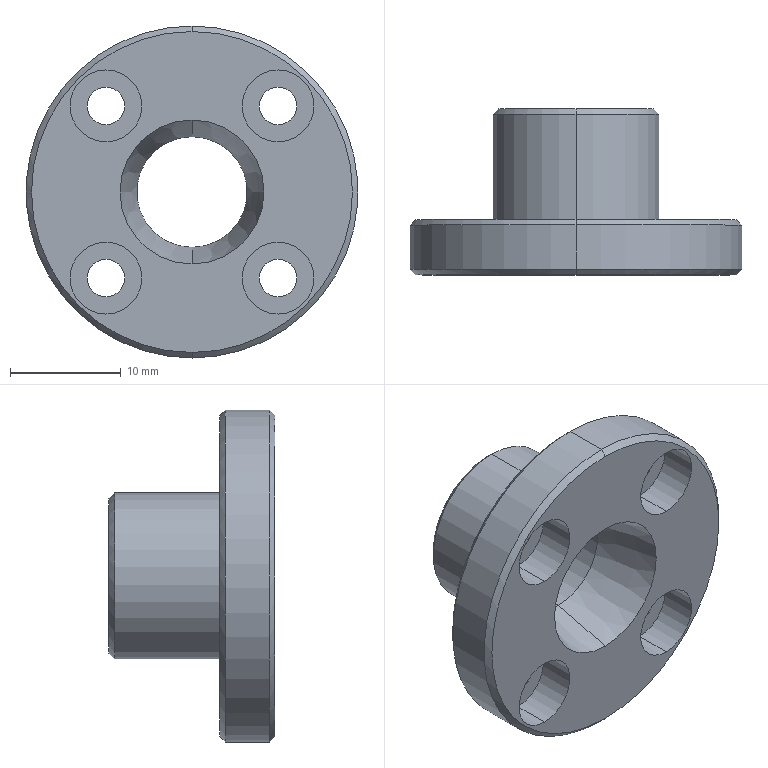Component | SolidWorks | SAWH02-03112A0LocatingBlock-1 | 1 solid | 37 faces | box 30 x 15 x 30 mm | volume 3429 mm3 | cylinder 22 | cone 8 | plane 7 | commonest cylinder face diameters 6.5 x8 3.4 x8 10 x2 15 x2 30 x2 | material 45
build123d program:
from build123d import *

# Parameters (mm, degrees)
M3_HEX_SOCKET_HEAD_CAP_SCREW_CBORE1_D           = 3.4
M3_HEX_SOCKET_HEAD_CAP_SCREW_CBORE1_DEPTH       = 12.4
M3_HEX_SOCKET_HEAD_CAP_SCREW_CBORE1_CBORE_D     = 6.5
M3_HEX_SOCKET_HEAD_CAP_SCREW_CBORE1_CBORE_DEPTH = 3.4
M3_HEX_SOCKET_HEAD_CAP_SCREW_CBORE1_TIP         = 1.021
CHAMFER1_SIZE                                   = 0.5


with BuildPart() as part:
    # Sketch1 → Revolve1 (revolve)
    with BuildSketch(Plane.XY, mode=Mode.PRIVATE) as revolve1_sk:
        Polygon((6.5, 0), (5, 6), (5, 15), (7.5, 15), (7.5, 5), (15, 5), (15, 0), align=None)
    revolve(revolve1_sk.sketch.rotate(Axis((0, 0, 0), (0, 1, 0)), 90), axis=Axis((0, 0, 0), (0, 1, 0)))

    # M3 Hex Socket Head Cap Screw CBORE1
    with Locations(Plane(origin=(0, 0, 0), x_dir=(-1, 0, 0), z_dir=(0, -1, 0))):
        with Locations((7.778, -7.778), (7.778, 7.778), (-7.778, 7.778), (-7.778, -7.778)):
            CounterBoreHole(M3_HEX_SOCKET_HEAD_CAP_SCREW_CBORE1_D / 2, M3_HEX_SOCKET_HEAD_CAP_SCREW_CBORE1_CBORE_D / 2, M3_HEX_SOCKET_HEAD_CAP_SCREW_CBORE1_CBORE_DEPTH, depth=M3_HEX_SOCKET_HEAD_CAP_SCREW_CBORE1_DEPTH)
            with Locations((0, 0, -(M3_HEX_SOCKET_HEAD_CAP_SCREW_CBORE1_DEPTH + M3_HEX_SOCKET_HEAD_CAP_SCREW_CBORE1_TIP / 2))):  # 118° drill point
                Cone(0, M3_HEX_SOCKET_HEAD_CAP_SCREW_CBORE1_D / 2, M3_HEX_SOCKET_HEAD_CAP_SCREW_CBORE1_TIP, mode=Mode.SUBTRACT)

    # Chamfer1
    chamfer1_edges = [part.edges().sort_by_distance(p)[0] for p in [
        (0, 15, 7.5),
        (0, 5, 15),
        (0, 0, 15),
    ]]
    chamfer(chamfer1_edges, length=CHAMFER1_SIZE)


solid = part.part

# Placed as in the assembly
solid = solid.moved(Location((113.51, -30.388, -4.792), (0, 0, 0)))
STEP:
#1=CARTESIAN_POINT('',(4.469,-1.196,-0.7595));
#2=VERTEX_POINT('',#1);
#3=CARTESIAN_POINT('',(4.469,-1.196,0.3822));
#4=VERTEX_POINT('',#3);
#5=CARTESIAN_POINT('',(4.469,-1.196,-0.1887));
#6=DIRECTION('',(0.,-1.,0.));
#7=DIRECTION('',(0.,0.,-1.));
#8=AXIS2_PLACEMENT_3D('',#5,#6,#7);
#9=CIRCLE('',#8,0.5709);
#10=EDGE_CURVE('',#2,#4,#9,.T.);
#11=ORIENTED_EDGE('',*,*,#10,.F.);
#12=CARTESIAN_POINT('',(4.469,-1.177,-0.7792));
#13=VERTEX_POINT('',#12);
#14=CARTESIAN_POINT('',(4.469,-1.196,-0.7595));
#15=DIRECTION('',(0.,0.7071,-0.7071));
#16=VECTOR('',#15,39.37);
#17=LINE('',#14,#16);
#18=EDGE_CURVE('',#2,#13,#17,.T.);
#19=ORIENTED_EDGE('',*,*,#18,.T.);
#20=CARTESIAN_POINT('',(4.469,-1.177,0.4019));
#21=VERTEX_POINT('',#20);
#22=CARTESIAN_POINT('',(4.469,-1.177,-0.1887));
#23=DIRECTION('',(0.,1.,0.));
#24=DIRECTION('',(0.,0.,-1.));
#25=AXIS2_PLACEMENT_3D('',#22,#23,#24);
#26=CIRCLE('',#25,0.5906);
#27=EDGE_CURVE('',#21,#13,#26,.T.);
#28=ORIENTED_EDGE('',*,*,#27,.F.);
#29=CARTESIAN_POINT('',(4.469,-1.196,0.3822));
#30=DIRECTION('',(0.,0.7071,0.7071));
#31=VECTOR('',#30,39.37);
#32=LINE('',#29,#31);
#33=EDGE_CURVE('',#4,#21,#32,.T.);
#34=ORIENTED_EDGE('',*,*,#33,.F.);
#35=EDGE_LOOP('',(#11,#19,#28,#34));
#36=FACE_OUTER_BOUND('',#35,.T.);
#37=CARTESIAN_POINT('',(4.469,-1.196,-0.1887));
#38=DIRECTION('',(0.,1.,0.));
#39=DIRECTION('',(0.,0.,1.));
#40=AXIS2_PLACEMENT_3D('',#37,#38,#39);
#41=CONICAL_SURFACE('',#40,0.5709,0.7854);
#42=ADVANCED_FACE('',(#36),#41,.T.);
#43=CARTESIAN_POINT('',(4.469,-0.9995,0.3822));
#44=VERTEX_POINT('',#43);
#45=CARTESIAN_POINT('',(4.469,-0.9995,-0.7595));
#46=VERTEX_POINT('',#45);
#47=CARTESIAN_POINT('',(4.469,-0.9995,-0.1887));
#48=DIRECTION('',(0.,1.,0.));
#49=DIRECTION('',(0.,0.,1.));
#50=AXIS2_PLACEMENT_3D('',#47,#48,#49);
#51=CIRCLE('',#50,0.5709);
#52=EDGE_CURVE('',#44,#46,#51,.T.);
#53=ORIENTED_EDGE('',*,*,#52,.F.);
#54=CARTESIAN_POINT('',(4.469,-1.019,0.4019));
#55=VERTEX_POINT('',#54);
#56=CARTESIAN_POINT('',(4.469,-1.019,0.4019));
#57=DIRECTION('',(0.,-0.7071,0.7071));
#58=VECTOR('',#57,39.37);
#59=LINE('',#56,#58);
#60=EDGE_CURVE('',#44,#55,#59,.T.);
#61=ORIENTED_EDGE('',*,*,#60,.T.);
#62=CARTESIAN_POINT('',(4.469,-1.019,-0.7792));
#63=VERTEX_POINT('',#62);
#64=CARTESIAN_POINT('',(4.469,-1.019,-0.1887));
#65=DIRECTION('',(0.,-1.,0.));
#66=DIRECTION('',(0.,0.,1.));
#67=AXIS2_PLACEMENT_3D('',#64,#65,#66);
#68=CIRCLE('',#67,0.5906);
#69=EDGE_CURVE('',#63,#55,#68,.T.);
#70=ORIENTED_EDGE('',*,*,#69,.F.);
#71=CARTESIAN_POINT('',(4.469,-1.019,-0.7792));
#72=DIRECTION('',(0.,-0.7071,-0.7071));
#73=VECTOR('',#72,39.37);
#74=LINE('',#71,#73);
#75=EDGE_CURVE('',#46,#63,#74,.T.);
#76=ORIENTED_EDGE('',*,*,#75,.F.);
#77=EDGE_LOOP('',(#53,#61,#70,#76));
#78=FACE_OUTER_BOUND('',#77,.T.);
#79=CARTESIAN_POINT('',(4.469,-1.019,-0.1887));
#80=DIRECTION('',(0.,-1.,0.));
#81=DIRECTION('',(0.,0.,-1.));
#82=AXIS2_PLACEMENT_3D('',#79,#80,#81);
#83=CONICAL_SURFACE('',#82,0.5906,0.7854);
#84=ADVANCED_FACE('',(#78),#83,.T.);
#85=CARTESIAN_POINT('',(4.469,-0.6058,0.08692));
#86=VERTEX_POINT('',#85);
#87=CARTESIAN_POINT('',(4.469,-0.6058,-0.4643));
#88=VERTEX_POINT('',#87);
#89=CARTESIAN_POINT('',(4.469,-0.6058,-0.1887));
#90=DIRECTION('',(0.,1.,0.));
#91=DIRECTION('',(0.,0.,1.));
#92=AXIS2_PLACEMENT_3D('',#89,#90,#91);
#93=CIRCLE('',#92,0.2756);
#94=EDGE_CURVE('',#86,#88,#93,.T.);
#95=ORIENTED_EDGE('',*,*,#94,.F.);
#96=CARTESIAN_POINT('',(4.469,-0.6255,0.1066));
#97=VERTEX_POINT('',#96);
#98=CARTESIAN_POINT('',(4.469,-0.6255,0.1066));
#99=DIRECTION('',(0.,-0.7071,0.7071));
#100=VECTOR('',#99,39.37);
#101=LINE('',#98,#100);
#102=EDGE_CURVE('',#86,#97,#101,.T.);
#103=ORIENTED_EDGE('',*,*,#102,.T.);
#104=CARTESIAN_POINT('',(4.469,-0.6255,-0.4839));
#105=VERTEX_POINT('',#104);
#106=CARTESIAN_POINT('',(4.469,-0.6255,-0.1887));
#107=DIRECTION('',(0.,-1.,0.));
#108=DIRECTION('',(0.,0.,1.));
#109=AXIS2_PLACEMENT_3D('',#106,#107,#108);
#110=CIRCLE('',#109,0.2953);
#111=EDGE_CURVE('',#105,#97,#110,.T.);
#112=ORIENTED_EDGE('',*,*,#111,.F.);
#113=CARTESIAN_POINT('',(4.469,-0.6255,-0.4839));
#114=DIRECTION('',(0.,-0.7071,-0.7071));
#115=VECTOR('',#114,39.37);
#116=LINE('',#113,#115);
#117=EDGE_CURVE('',#88,#105,#116,.T.);
#118=ORIENTED_EDGE('',*,*,#117,.F.);
#119=EDGE_LOOP('',(#95,#103,#112,#118));
#120=FACE_OUTER_BOUND('',#119,.T.);
#121=CARTESIAN_POINT('',(4.469,-0.6255,-0.1887));
#122=DIRECTION('',(0.,-1.,0.));
#123=DIRECTION('',(0.,0.,-1.));
#124=AXIS2_PLACEMENT_3D('',#121,#122,#123);
#125=CONICAL_SURFACE('',#124,0.2953,0.7854);
#126=ADVANCED_FACE('',(#120),#125,.T.);
#127=CARTESIAN_POINT('',(4.163,-1.063,0.2455));
#128=VERTEX_POINT('',#127);
#129=CARTESIAN_POINT('',(4.163,-1.063,-0.01039));
#130=VERTEX_POINT('',#129);
#131=CARTESIAN_POINT('',(4.163,-1.063,0.1176));
#132=DIRECTION('',(0.,-1.,0.));
#133=DIRECTION('',(0.,0.,-1.));
#134=AXIS2_PLACEMENT_3D('',#131,#132,#133);
#135=CIRCLE('',#134,0.128);
#136=EDGE_CURVE('',#128,#130,#135,.T.);
#137=ORIENTED_EDGE('',*,*,#136,.F.);
#138=CARTESIAN_POINT('',(4.163,-1.196,0.2455));
#139=VERTEX_POINT('',#138);
#140=CARTESIAN_POINT('',(4.163,-1.196,0.2455));
#141=DIRECTION('',(0.,-1.,0.));
#142=VECTOR('',#141,39.37);
#143=LINE('',#140,#142);
#144=EDGE_CURVE('',#128,#139,#143,.T.);
#145=ORIENTED_EDGE('',*,*,#144,.T.);
#146=CARTESIAN_POINT('',(4.163,-1.196,-0.01039));
#147=VERTEX_POINT('',#146);
#148=CARTESIAN_POINT('',(4.163,-1.196,0.1176));
#149=DIRECTION('',(0.,-1.,0.));
#150=DIRECTION('',(0.,0.,-1.));
#151=AXIS2_PLACEMENT_3D('',#148,#149,#150);
#152=CIRCLE('',#151,0.128);
#153=EDGE_CURVE('',#139,#147,#152,.T.);
#154=ORIENTED_EDGE('',*,*,#153,.T.);
#155=CARTESIAN_POINT('',(4.163,-1.196,-0.01039));
#156=DIRECTION('',(0.,-1.,0.));
#157=VECTOR('',#156,39.37);
#158=LINE('',#155,#157);
#159=EDGE_CURVE('',#130,#147,#158,.T.);
#160=ORIENTED_EDGE('',*,*,#159,.F.);
#161=EDGE_LOOP('',(#137,#145,#154,#160));
#162=FACE_OUTER_BOUND('',#161,.T.);
#163=CARTESIAN_POINT('',(4.163,-1.196,0.1176));
#164=DIRECTION('',(0.,-1.,0.));
#165=DIRECTION('',(0.,0.,-1.));
#166=AXIS2_PLACEMENT_3D('',#163,#164,#165);
#167=CYLINDRICAL_SURFACE('',#166,0.128);
#168=ADVANCED_FACE('',(#162),#167,.F.);
#169=CARTESIAN_POINT('',(4.163,-0.9995,0.05063));
#170=VERTEX_POINT('',#169);
#171=CARTESIAN_POINT('',(4.163,-0.9995,0.1845));
#172=VERTEX_POINT('',#171);
#173=CARTESIAN_POINT('',(4.163,-0.9995,0.1176));
#174=DIRECTION('',(0.,1.,0.));
#175=DIRECTION('',(0.,0.,1.));
#176=AXIS2_PLACEMENT_3D('',#173,#174,#175);
#177=CIRCLE('',#176,0.06693);
#178=EDGE_CURVE('',#170,#172,#177,.T.);
#179=ORIENTED_EDGE('',*,*,#178,.T.);
#180=CARTESIAN_POINT('',(4.163,-1.063,0.1845));
#181=VERTEX_POINT('',#180);
#182=CARTESIAN_POINT('',(4.163,-1.196,0.1845));
#183=DIRECTION('',(0.,-1.,0.));
#184=VECTOR('',#183,39.37);
#185=LINE('',#182,#184);
#186=EDGE_CURVE('',#172,#181,#185,.T.);
#187=ORIENTED_EDGE('',*,*,#186,.T.);
#188=CARTESIAN_POINT('',(4.163,-1.063,0.05063));
#189=VERTEX_POINT('',#188);
#190=CARTESIAN_POINT('',(4.163,-1.063,0.1176));
#191=DIRECTION('',(0.,-1.,0.));
#192=DIRECTION('',(0.,0.,-1.));
#193=AXIS2_PLACEMENT_3D('',#190,#191,#192);
#194=CIRCLE('',#193,0.06693);
#195=EDGE_CURVE('',#181,#189,#194,.T.);
#196=ORIENTED_EDGE('',*,*,#195,.T.);
#197=CARTESIAN_POINT('',(4.163,-1.196,0.05063));
#198=DIRECTION('',(0.,-1.,0.));
#199=VECTOR('',#198,39.37);
#200=LINE('',#197,#199);
#201=EDGE_CURVE('',#170,#189,#200,.T.);
#202=ORIENTED_EDGE('',*,*,#201,.F.);
#203=EDGE_LOOP('',(#179,#187,#196,#202));
#204=FACE_OUTER_BOUND('',#203,.T.);
#205=CARTESIAN_POINT('',(4.163,-1.196,0.1176));
#206=DIRECTION('',(0.,-1.,0.));
#207=DIRECTION('',(0.,0.,-1.));
#208=AXIS2_PLACEMENT_3D('',#205,#206,#207);
#209=CYLINDRICAL_SURFACE('',#208,0.06693);
#210=ADVANCED_FACE('',(#204),#209,.F.);
#211=CARTESIAN_POINT('',(4.163,-1.063,-0.3669));
#212=VERTEX_POINT('',#211);
#213=CARTESIAN_POINT('',(4.163,-1.063,-0.6228));
#214=VERTEX_POINT('',#213);
#215=CARTESIAN_POINT('',(4.163,-1.063,-0.4949));
#216=DIRECTION('',(0.,-1.,0.));
#217=DIRECTION('',(0.,0.,-1.));
#218=AXIS2_PLACEMENT_3D('',#215,#216,#217);
#219=CIRCLE('',#218,0.128);
#220=EDGE_CURVE('',#212,#214,#219,.T.);
#221=ORIENTED_EDGE('',*,*,#220,.F.);
#222=CARTESIAN_POINT('',(4.163,-1.196,-0.3669));
#223=VERTEX_POINT('',#222);
#224=CARTESIAN_POINT('',(4.163,-1.196,-0.3669));
#225=DIRECTION('',(0.,-1.,0.));
#226=VECTOR('',#225,39.37);
#227=LINE('',#224,#226);
#228=EDGE_CURVE('',#212,#223,#227,.T.);
#229=ORIENTED_EDGE('',*,*,#228,.T.);
#230=CARTESIAN_POINT('',(4.163,-1.196,-0.6228));
#231=VERTEX_POINT('',#230);
#232=CARTESIAN_POINT('',(4.163,-1.196,-0.4949));
#233=DIRECTION('',(0.,-1.,0.));
#234=DIRECTION('',(0.,0.,-1.));
#235=AXIS2_PLACEMENT_3D('',#232,#233,#234);
#236=CIRCLE('',#235,0.128);
#237=EDGE_CURVE('',#223,#231,#236,.T.);
#238=ORIENTED_EDGE('',*,*,#237,.T.);
#239=CARTESIAN_POINT('',(4.163,-1.196,-0.6228));
#240=DIRECTION('',(0.,-1.,0.));
#241=VECTOR('',#240,39.37);
#242=LINE('',#239,#241);
#243=EDGE_CURVE('',#214,#231,#242,.T.);
#244=ORIENTED_EDGE('',*,*,#243,.F.);
#245=EDGE_LOOP('',(#221,#229,#238,#244));
#246=FACE_OUTER_BOUND('',#245,.T.);
#247=CARTESIAN_POINT('',(4.163,-1.196,-0.4949));
#248=DIRECTION('',(0.,-1.,0.));
#249=DIRECTION('',(0.,0.,-1.));
#250=AXIS2_PLACEMENT_3D('',#247,#248,#249);
#251=CYLINDRICAL_SURFACE('',#250,0.128);
#252=ADVANCED_FACE('',(#246),#251,.F.);
#253=CARTESIAN_POINT('',(4.163,-0.9995,-0.5618));
#254=VERTEX_POINT('',#253);
#255=CARTESIAN_POINT('',(4.163,-0.9995,-0.428));
#256=VERTEX_POINT('',#255);
#257=CARTESIAN_POINT('',(4.163,-0.9995,-0.4949));
#258=DIRECTION('',(0.,1.,0.));
#259=DIRECTION('',(0.,0.,1.));
#260=AXIS2_PLACEMENT_3D('',#257,#258,#259);
#261=CIRCLE('',#260,0.06693);
#262=EDGE_CURVE('',#254,#256,#261,.T.);
#263=ORIENTED_EDGE('',*,*,#262,.T.);
#264=CARTESIAN_POINT('',(4.163,-1.063,-0.428));
#265=VERTEX_POINT('',#264);
#266=CARTESIAN_POINT('',(4.163,-1.196,-0.428));
#267=DIRECTION('',(0.,-1.,0.));
#268=VECTOR('',#267,39.37);
#269=LINE('',#266,#268);
#270=EDGE_CURVE('',#256,#265,#269,.T.);
#271=ORIENTED_EDGE('',*,*,#270,.T.);
#272=CARTESIAN_POINT('',(4.163,-1.063,-0.5618));
#273=VERTEX_POINT('',#272);
#274=CARTESIAN_POINT('',(4.163,-1.063,-0.4949));
#275=DIRECTION('',(0.,-1.,0.));
#276=DIRECTION('',(0.,0.,-1.));
#277=AXIS2_PLACEMENT_3D('',#274,#275,#276);
#278=CIRCLE('',#277,0.06693);
#279=EDGE_CURVE('',#265,#273,#278,.T.);
#280=ORIENTED_EDGE('',*,*,#279,.T.);
#281=CARTESIAN_POINT('',(4.163,-1.196,-0.5618));
#282=DIRECTION('',(0.,-1.,0.));
#283=VECTOR('',#282,39.37);
#284=LINE('',#281,#283);
#285=EDGE_CURVE('',#254,#273,#284,.T.);
#286=ORIENTED_EDGE('',*,*,#285,.F.);
#287=EDGE_LOOP('',(#263,#271,#280,#286));
#288=FACE_OUTER_BOUND('',#287,.T.);
#289=CARTESIAN_POINT('',(4.163,-1.196,-0.4949));
#290=DIRECTION('',(0.,-1.,0.));
#291=DIRECTION('',(0.,0.,-1.));
#292=AXIS2_PLACEMENT_3D('',#289,#290,#291);
#293=CYLINDRICAL_SURFACE('',#292,0.06693);
#294=ADVANCED_FACE('',(#288),#293,.F.);
#295=CARTESIAN_POINT('',(4.775,-1.063,-0.3669));
#296=VERTEX_POINT('',#295);
#297=CARTESIAN_POINT('',(4.775,-1.063,-0.6228));
#298=VERTEX_POINT('',#297);
#299=CARTESIAN_POINT('',(4.775,-1.063,-0.4949));
#300=DIRECTION('',(0.,-1.,0.));
#301=DIRECTION('',(0.,0.,-1.));
#302=AXIS2_PLACEMENT_3D('',#299,#300,#301);
#303=CIRCLE('',#302,0.128);
#304=EDGE_CURVE('',#296,#298,#303,.T.);
#305=ORIENTED_EDGE('',*,*,#304,.F.);
#306=CARTESIAN_POINT('',(4.775,-1.196,-0.3669));
#307=VERTEX_POINT('',#306);
#308=CARTESIAN_POINT('',(4.775,-1.196,-0.3669));
#309=DIRECTION('',(0.,-1.,0.));
#310=VECTOR('',#309,39.37);
#311=LINE('',#308,#310);
#312=EDGE_CURVE('',#296,#307,#311,.T.);
#313=ORIENTED_EDGE('',*,*,#312,.T.);
#314=CARTESIAN_POINT('',(4.775,-1.196,-0.6228));
#315=VERTEX_POINT('',#314);
#316=CARTESIAN_POINT('',(4.775,-1.196,-0.4949));
#317=DIRECTION('',(0.,-1.,0.));
#318=DIRECTION('',(0.,0.,-1.));
#319=AXIS2_PLACEMENT_3D('',#316,#317,#318);
#320=CIRCLE('',#319,0.128);
#321=EDGE_CURVE('',#307,#315,#320,.T.);
#322=ORIENTED_EDGE('',*,*,#321,.T.);
#323=CARTESIAN_POINT('',(4.775,-1.196,-0.6228));
#324=DIRECTION('',(0.,-1.,0.));
#325=VECTOR('',#324,39.37);
#326=LINE('',#323,#325);
#327=EDGE_CURVE('',#298,#315,#326,.T.);
#328=ORIENTED_EDGE('',*,*,#327,.F.);
#329=EDGE_LOOP('',(#305,#313,#322,#328));
#330=FACE_OUTER_BOUND('',#329,.T.);
#331=CARTESIAN_POINT('',(4.775,-1.196,-0.4949));
#332=DIRECTION('',(0.,-1.,0.));
#333=DIRECTION('',(0.,0.,-1.));
#334=AXIS2_PLACEMENT_3D('',#331,#332,#333);
#335=CYLINDRICAL_SURFACE('',#334,0.128);
#336=ADVANCED_FACE('',(#330),#335,.F.);
#337=CARTESIAN_POINT('',(4.775,-0.9995,-0.5618));
#338=VERTEX_POINT('',#337);
#339=CARTESIAN_POINT('',(4.775,-0.9995,-0.428));
#340=VERTEX_POINT('',#339);
#341=CARTESIAN_POINT('',(4.775,-0.9995,-0.4949));
#342=DIRECTION('',(0.,1.,0.));
#343=DIRECTION('',(0.,0.,1.));
#344=AXIS2_PLACEMENT_3D('',#341,#342,#343);
#345=CIRCLE('',#344,0.06693);
#346=EDGE_CURVE('',#338,#340,#345,.T.);
#347=ORIENTED_EDGE('',*,*,#346,.T.);
#348=CARTESIAN_POINT('',(4.775,-1.063,-0.428));
#349=VERTEX_POINT('',#348);
#350=CARTESIAN_POINT('',(4.775,-1.196,-0.428));
#351=DIRECTION('',(0.,-1.,0.));
#352=VECTOR('',#351,39.37);
#353=LINE('',#350,#352);
#354=EDGE_CURVE('',#340,#349,#353,.T.);
#355=ORIENTED_EDGE('',*,*,#354,.T.);
#356=CARTESIAN_POINT('',(4.775,-1.063,-0.5618));
#357=VERTEX_POINT('',#356);
#358=CARTESIAN_POINT('',(4.775,-1.063,-0.4949));
#359=DIRECTION('',(0.,-1.,0.));
#360=DIRECTION('',(0.,0.,-1.));
#361=AXIS2_PLACEMENT_3D('',#358,#359,#360);
#362=CIRCLE('',#361,0.06693);
#363=EDGE_CURVE('',#349,#357,#362,.T.);
#364=ORIENTED_EDGE('',*,*,#363,.T.);
#365=CARTESIAN_POINT('',(4.775,-1.196,-0.5618));
#366=DIRECTION('',(0.,-1.,0.));
#367=VECTOR('',#366,39.37);
#368=LINE('',#365,#367);
#369=EDGE_CURVE('',#338,#357,#368,.T.);
#370=ORIENTED_EDGE('',*,*,#369,.F.);
#371=EDGE_LOOP('',(#347,#355,#364,#370));
#372=FACE_OUTER_BOUND('',#371,.T.);
#373=CARTESIAN_POINT('',(4.775,-1.196,-0.4949));
#374=DIRECTION('',(0.,-1.,0.));
#375=DIRECTION('',(0.,0.,-1.));
#376=AXIS2_PLACEMENT_3D('',#373,#374,#375);
#377=CYLINDRICAL_SURFACE('',#376,0.06693);
#378=ADVANCED_FACE('',(#372),#377,.F.);
#379=CARTESIAN_POINT('',(4.775,-1.063,0.2455));
#380=VERTEX_POINT('',#379);
#381=CARTESIAN_POINT('',(4.775,-1.063,-0.01039));
#382=VERTEX_POINT('',#381);
#383=CARTESIAN_POINT('',(4.775,-1.063,0.1176));
#384=DIRECTION('',(0.,-1.,0.));
#385=DIRECTION('',(0.,0.,-1.));
#386=AXIS2_PLACEMENT_3D('',#383,#384,#385);
#387=CIRCLE('',#386,0.128);
#388=EDGE_CURVE('',#380,#382,#387,.T.);
#389=ORIENTED_EDGE('',*,*,#388,.F.);
#390=CARTESIAN_POINT('',(4.775,-1.196,0.2455));
#391=VERTEX_POINT('',#390);
#392=CARTESIAN_POINT('',(4.775,-1.196,0.2455));
#393=DIRECTION('',(0.,-1.,0.));
#394=VECTOR('',#393,39.37);
#395=LINE('',#392,#394);
#396=EDGE_CURVE('',#380,#391,#395,.T.);
#397=ORIENTED_EDGE('',*,*,#396,.T.);
#398=CARTESIAN_POINT('',(4.775,-1.196,-0.01039));
#399=VERTEX_POINT('',#398);
#400=CARTESIAN_POINT('',(4.775,-1.196,0.1176));
#401=DIRECTION('',(0.,-1.,0.));
#402=DIRECTION('',(0.,0.,-1.));
#403=AXIS2_PLACEMENT_3D('',#400,#401,#402);
#404=CIRCLE('',#403,0.128);
#405=EDGE_CURVE('',#391,#399,#404,.T.);
#406=ORIENTED_EDGE('',*,*,#405,.T.);
#407=CARTESIAN_POINT('',(4.775,-1.196,-0.01039));
#408=DIRECTION('',(0.,-1.,0.));
#409=VECTOR('',#408,39.37);
#410=LINE('',#407,#409);
#411=EDGE_CURVE('',#382,#399,#410,.T.);
#412=ORIENTED_EDGE('',*,*,#411,.F.);
#413=EDGE_LOOP('',(#389,#397,#406,#412));
#414=FACE_OUTER_BOUND('',#413,.T.);
#415=CARTESIAN_POINT('',(4.775,-1.196,0.1176));
#416=DIRECTION('',(0.,-1.,0.));
#417=DIRECTION('',(0.,0.,-1.));
#418=AXIS2_PLACEMENT_3D('',#415,#416,#417);
#419=CYLINDRICAL_SURFACE('',#418,0.128);
#420=ADVANCED_FACE('',(#414),#419,.F.);
#421=CARTESIAN_POINT('',(4.775,-0.9995,0.05063));
#422=VERTEX_POINT('',#421);
#423=CARTESIAN_POINT('',(4.775,-0.9995,0.1845));
#424=VERTEX_POINT('',#423);
#425=CARTESIAN_POINT('',(4.775,-0.9995,0.1176));
#426=DIRECTION('',(0.,1.,0.));
#427=DIRECTION('',(0.,0.,1.));
#428=AXIS2_PLACEMENT_3D('',#425,#426,#427);
#429=CIRCLE('',#428,0.06693);
#430=EDGE_CURVE('',#422,#424,#429,.T.);
#431=ORIENTED_EDGE('',*,*,#430,.T.);
#432=CARTESIAN_POINT('',(4.775,-1.063,0.1845));
#433=VERTEX_POINT('',#432);
#434=CARTESIAN_POINT('',(4.775,-1.196,0.1845));
#435=DIRECTION('',(0.,-1.,0.));
#436=VECTOR('',#435,39.37);
#437=LINE('',#434,#436);
#438=EDGE_CURVE('',#424,#433,#437,.T.);
#439=ORIENTED_EDGE('',*,*,#438,.T.);
#440=CARTESIAN_POINT('',(4.775,-1.063,0.05063));
#441=VERTEX_POINT('',#440);
#442=CARTESIAN_POINT('',(4.775,-1.063,0.1176));
#443=DIRECTION('',(0.,-1.,0.));
#444=DIRECTION('',(0.,0.,-1.));
#445=AXIS2_PLACEMENT_3D('',#442,#443,#444);
#446=CIRCLE('',#445,0.06693);
#447=EDGE_CURVE('',#433,#441,#446,.T.);
#448=ORIENTED_EDGE('',*,*,#447,.T.);
#449=CARTESIAN_POINT('',(4.775,-1.196,0.05063));
#450=DIRECTION('',(0.,-1.,0.));
#451=VECTOR('',#450,39.37);
#452=LINE('',#449,#451);
#453=EDGE_CURVE('',#422,#441,#452,.T.);
#454=ORIENTED_EDGE('',*,*,#453,.F.);
#455=EDGE_LOOP('',(#431,#439,#448,#454));
#456=FACE_OUTER_BOUND('',#455,.T.);
#457=CARTESIAN_POINT('',(4.775,-1.196,0.1176));
#458=DIRECTION('',(0.,-1.,0.));
#459=DIRECTION('',(0.,0.,-1.));
#460=AXIS2_PLACEMENT_3D('',#457,#458,#459);
#461=CYLINDRICAL_SURFACE('',#460,0.06693);
#462=ADVANCED_FACE('',(#456),#461,.F.);
#463=CARTESIAN_POINT('',(4.469,-0.9601,0.008181));
#464=VERTEX_POINT('',#463);
#465=CARTESIAN_POINT('',(4.469,-0.9601,-0.3855));
#466=VERTEX_POINT('',#465);
#467=CARTESIAN_POINT('',(4.469,-0.9601,-0.1887));
#468=DIRECTION('',(0.,-1.,0.));
#469=DIRECTION('',(0.,0.,-1.));
#470=AXIS2_PLACEMENT_3D('',#467,#468,#469);
#471=CIRCLE('',#470,0.1969);
#472=EDGE_CURVE('',#464,#466,#471,.T.);
#473=ORIENTED_EDGE('',*,*,#472,.F.);
#474=CARTESIAN_POINT('',(4.469,-1.196,0.06724));
#475=VERTEX_POINT('',#474);
#476=CARTESIAN_POINT('',(4.469,-0.9601,0.008181));
#477=DIRECTION('',(0.,-0.9701,0.2425));
#478=VECTOR('',#477,39.37);
#479=LINE('',#476,#478);
#480=EDGE_CURVE('',#464,#475,#479,.T.);
#481=ORIENTED_EDGE('',*,*,#480,.T.);
#482=CARTESIAN_POINT('',(4.469,-1.196,-0.4446));
#483=VERTEX_POINT('',#482);
#484=CARTESIAN_POINT('',(4.469,-1.196,-0.1887));
#485=DIRECTION('',(0.,-1.,0.));
#486=DIRECTION('',(0.,0.,-1.));
#487=AXIS2_PLACEMENT_3D('',#484,#485,#486);
#488=CIRCLE('',#487,0.2559);
#489=EDGE_CURVE('',#475,#483,#488,.T.);
#490=ORIENTED_EDGE('',*,*,#489,.T.);
#491=CARTESIAN_POINT('',(4.469,-0.9601,-0.3855));
#492=DIRECTION('',(0.,-0.9701,-0.2425));
#493=VECTOR('',#492,39.37);
#494=LINE('',#491,#493);
#495=EDGE_CURVE('',#466,#483,#494,.T.);
#496=ORIENTED_EDGE('',*,*,#495,.F.);
#497=EDGE_LOOP('',(#473,#481,#490,#496));
#498=FACE_OUTER_BOUND('',#497,.T.);
#499=CARTESIAN_POINT('',(4.469,-0.9601,-0.1887));
#500=DIRECTION('',(0.,-1.,0.));
#501=DIRECTION('',(0.,0.,-1.));
#502=AXIS2_PLACEMENT_3D('',#499,#500,#501);
#503=CONICAL_SURFACE('',#502,0.1969,0.245);
#504=ADVANCED_FACE('',(#498),#503,.F.);
#505=CARTESIAN_POINT('',(4.469,-0.6058,0.008181));
#506=VERTEX_POINT('',#505);
#507=CARTESIAN_POINT('',(4.469,-0.6058,-0.3855));
#508=VERTEX_POINT('',#507);
#509=CARTESIAN_POINT('',(4.469,-0.6058,-0.1887));
#510=DIRECTION('',(0.,-1.,0.));
#511=DIRECTION('',(0.,0.,-1.));
#512=AXIS2_PLACEMENT_3D('',#509,#510,#511);
#513=CIRCLE('',#512,0.1969);
#514=EDGE_CURVE('',#506,#508,#513,.T.);
#515=ORIENTED_EDGE('',*,*,#514,.F.);
#516=CARTESIAN_POINT('',(4.469,-1.196,0.008181));
#517=DIRECTION('',(0.,-1.,0.));
#518=VECTOR('',#517,39.37);
#519=LINE('',#516,#518);
#520=EDGE_CURVE('',#506,#464,#519,.T.);
#521=ORIENTED_EDGE('',*,*,#520,.T.);
#522=ORIENTED_EDGE('',*,*,#472,.T.);
#523=CARTESIAN_POINT('',(4.469,-1.196,-0.3855));
#524=DIRECTION('',(0.,-1.,0.));
#525=VECTOR('',#524,39.37);
#526=LINE('',#523,#525);
#527=EDGE_CURVE('',#508,#466,#526,.T.);
#528=ORIENTED_EDGE('',*,*,#527,.F.);
#529=EDGE_LOOP('',(#515,#521,#522,#528));
#530=FACE_OUTER_BOUND('',#529,.T.);
#531=CARTESIAN_POINT('',(4.469,-1.196,-0.1887));
#532=DIRECTION('',(0.,-1.,0.));
#533=DIRECTION('',(0.,0.,-1.));
#534=AXIS2_PLACEMENT_3D('',#531,#532,#533);
#535=CYLINDRICAL_SURFACE('',#534,0.1969);
#536=ADVANCED_FACE('',(#530),#535,.F.);
#537=ORIENTED_EDGE('',*,*,#111,.T.);
#538=CARTESIAN_POINT('',(4.469,-0.9995,0.1066));
#539=VERTEX_POINT('',#538);
#540=CARTESIAN_POINT('',(4.469,-1.196,0.1066));
#541=DIRECTION('',(0.,-1.,0.));
#542=VECTOR('',#541,39.37);
#543=LINE('',#540,#542);
#544=EDGE_CURVE('',#97,#539,#543,.T.);
#545=ORIENTED_EDGE('',*,*,#544,.T.);
#546=CARTESIAN_POINT('',(4.469,-0.9995,-0.4839));
#547=VERTEX_POINT('',#546);
#548=CARTESIAN_POINT('',(4.469,-0.9995,-0.1887));
#549=DIRECTION('',(0.,-1.,0.));
#550=DIRECTION('',(0.,0.,-1.));
#551=AXIS2_PLACEMENT_3D('',#548,#549,#550);
#552=CIRCLE('',#551,0.2953);
#553=EDGE_CURVE('',#547,#539,#552,.T.);
#554=ORIENTED_EDGE('',*,*,#553,.F.);
#555=CARTESIAN_POINT('',(4.469,-1.196,-0.4839));
#556=DIRECTION('',(0.,-1.,0.));
#557=VECTOR('',#556,39.37);
#558=LINE('',#555,#557);
#559=EDGE_CURVE('',#105,#547,#558,.T.);
#560=ORIENTED_EDGE('',*,*,#559,.F.);
#561=EDGE_LOOP('',(#537,#545,#554,#560));
#562=FACE_OUTER_BOUND('',#561,.T.);
#563=CARTESIAN_POINT('',(4.469,-1.196,-0.1887));
#564=DIRECTION('',(0.,-1.,0.));
#565=DIRECTION('',(0.,0.,-1.));
#566=AXIS2_PLACEMENT_3D('',#563,#564,#565);
#567=CYLINDRICAL_SURFACE('',#566,0.2953);
#568=ADVANCED_FACE('',(#562),#567,.T.);
#569=ORIENTED_EDGE('',*,*,#69,.T.);
#570=CARTESIAN_POINT('',(4.469,-1.196,0.4019));
#571=DIRECTION('',(0.,-1.,0.));
#572=VECTOR('',#571,39.37);
#573=LINE('',#570,#572);
#574=EDGE_CURVE('',#55,#21,#573,.T.);
#575=ORIENTED_EDGE('',*,*,#574,.T.);
#576=ORIENTED_EDGE('',*,*,#27,.T.);
#577=CARTESIAN_POINT('',(4.469,-1.196,-0.7792));
#578=DIRECTION('',(0.,-1.,0.));
#579=VECTOR('',#578,39.37);
#580=LINE('',#577,#579);
#581=EDGE_CURVE('',#63,#13,#580,.T.);
#582=ORIENTED_EDGE('',*,*,#581,.F.);
#583=EDGE_LOOP('',(#569,#575,#576,#582));
#584=FACE_OUTER_BOUND('',#583,.T.);
#585=CARTESIAN_POINT('',(4.469,-1.196,-0.1887));
#586=DIRECTION('',(0.,-1.,0.));
#587=DIRECTION('',(0.,0.,-1.));
#588=AXIS2_PLACEMENT_3D('',#585,#586,#587);
#589=CYLINDRICAL_SURFACE('',#588,0.5906);
#590=ADVANCED_FACE('',(#584),#589,.T.);
#591=CARTESIAN_POINT('',(4.469,-1.196,-0.1887));
#592=DIRECTION('',(0.,-1.,0.));
#593=DIRECTION('',(0.,0.,-1.));
#594=AXIS2_PLACEMENT_3D('',#591,#592,#593);
#595=CIRCLE('',#594,0.5709);
#596=EDGE_CURVE('',#4,#2,#595,.T.);
#597=ORIENTED_EDGE('',*,*,#596,.T.);
#598=ORIENTED_EDGE('',*,*,#10,.T.);
#599=EDGE_LOOP('',(#597,#598));
#600=FACE_OUTER_BOUND('',#599,.T.);
#601=CARTESIAN_POINT('',(4.163,-1.196,0.1176));
#602=DIRECTION('',(0.,-1.,0.));
#603=DIRECTION('',(0.,0.,-1.));
#604=AXIS2_PLACEMENT_3D('',#601,#602,#603);
#605=CIRCLE('',#604,0.128);
#606=EDGE_CURVE('',#147,#139,#605,.T.);
#607=ORIENTED_EDGE('',*,*,#606,.F.);
#608=ORIENTED_EDGE('',*,*,#153,.F.);
#609=EDGE_LOOP('',(#607,#608));
#610=FACE_BOUND('',#609,.T.);
#611=CARTESIAN_POINT('',(4.163,-1.196,-0.4949));
#612=DIRECTION('',(0.,-1.,0.));
#613=DIRECTION('',(0.,0.,-1.));
#614=AXIS2_PLACEMENT_3D('',#611,#612,#613);
#615=CIRCLE('',#614,0.128);
#616=EDGE_CURVE('',#231,#223,#615,.T.);
#617=ORIENTED_EDGE('',*,*,#616,.F.);
#618=ORIENTED_EDGE('',*,*,#237,.F.);
#619=EDGE_LOOP('',(#617,#618));
#620=FACE_BOUND('',#619,.T.);
#621=CARTESIAN_POINT('',(4.775,-1.196,-0.4949));
#622=DIRECTION('',(0.,-1.,0.));
#623=DIRECTION('',(0.,0.,-1.));
#624=AXIS2_PLACEMENT_3D('',#621,#622,#623);
#625=CIRCLE('',#624,0.128);
#626=EDGE_CURVE('',#315,#307,#625,.T.);
#627=ORIENTED_EDGE('',*,*,#626,.F.);
#628=ORIENTED_EDGE('',*,*,#321,.F.);
#629=EDGE_LOOP('',(#627,#628));
#630=FACE_BOUND('',#629,.T.);
#631=CARTESIAN_POINT('',(4.775,-1.196,0.1176));
#632=DIRECTION('',(0.,-1.,0.));
#633=DIRECTION('',(0.,0.,-1.));
#634=AXIS2_PLACEMENT_3D('',#631,#632,#633);
#635=CIRCLE('',#634,0.128);
#636=EDGE_CURVE('',#399,#391,#635,.T.);
#637=ORIENTED_EDGE('',*,*,#636,.F.);
#638=ORIENTED_EDGE('',*,*,#405,.F.);
#639=EDGE_LOOP('',(#637,#638));
#640=FACE_BOUND('',#639,.T.);
#641=CARTESIAN_POINT('',(4.469,-1.196,-0.1887));
#642=DIRECTION('',(0.,-1.,0.));
#643=DIRECTION('',(0.,0.,-1.));
#644=AXIS2_PLACEMENT_3D('',#641,#642,#643);
#645=CIRCLE('',#644,0.2559);
#646=EDGE_CURVE('',#483,#475,#645,.T.);
#647=ORIENTED_EDGE('',*,*,#646,.F.);
#648=ORIENTED_EDGE('',*,*,#489,.F.);
#649=EDGE_LOOP('',(#647,#648));
#650=FACE_BOUND('',#649,.T.);
#651=CARTESIAN_POINT('',(4.725,-1.196,-0.1887));
#652=DIRECTION('',(0.,-1.,0.));
#653=DIRECTION('',(0.,0.,-1.));
#654=AXIS2_PLACEMENT_3D('',#651,#652,#653);
#655=PLANE('',#654);
#656=ADVANCED_FACE('',(#600,#610,#620,#630,#640,#650),#655,.T.);
#657=ORIENTED_EDGE('',*,*,#574,.F.);
#658=CARTESIAN_POINT('',(4.469,-1.019,-0.1887));
#659=DIRECTION('',(0.,-1.,0.));
#660=DIRECTION('',(0.,0.,1.));
#661=AXIS2_PLACEMENT_3D('',#658,#659,#660);
#662=CIRCLE('',#661,0.5906);
#663=EDGE_CURVE('',#55,#63,#662,.T.);
#664=ORIENTED_EDGE('',*,*,#663,.T.);
#665=ORIENTED_EDGE('',*,*,#581,.T.);
#666=CARTESIAN_POINT('',(4.469,-1.177,-0.1887));
#667=DIRECTION('',(0.,1.,0.));
#668=DIRECTION('',(0.,0.,-1.));
#669=AXIS2_PLACEMENT_3D('',#666,#667,#668);
#670=CIRCLE('',#669,0.5906);
#671=EDGE_CURVE('',#13,#21,#670,.T.);
#672=ORIENTED_EDGE('',*,*,#671,.T.);
#673=EDGE_LOOP('',(#657,#664,#665,#672));
#674=FACE_OUTER_BOUND('',#673,.T.);
#675=CARTESIAN_POINT('',(4.469,-1.196,-0.1887));
#676=DIRECTION('',(0.,-1.,0.));
#677=DIRECTION('',(0.,0.,-1.));
#678=AXIS2_PLACEMENT_3D('',#675,#676,#677);
#679=CYLINDRICAL_SURFACE('',#678,0.5906);
#680=ADVANCED_FACE('',(#674),#679,.T.);
#681=CARTESIAN_POINT('',(4.469,-0.9995,-0.1887));
#682=DIRECTION('',(0.,1.,0.));
#683=DIRECTION('',(0.,0.,1.));
#684=AXIS2_PLACEMENT_3D('',#681,#682,#683);
#685=CIRCLE('',#684,0.5709);
#686=EDGE_CURVE('',#46,#44,#685,.T.);
#687=ORIENTED_EDGE('',*,*,#686,.T.);
#688=ORIENTED_EDGE('',*,*,#52,.T.);
#689=EDGE_LOOP('',(#687,#688));
#690=FACE_OUTER_BOUND('',#689,.T.);
#691=ORIENTED_EDGE('',*,*,#178,.F.);
#692=CARTESIAN_POINT('',(4.163,-0.9995,0.1176));
#693=DIRECTION('',(0.,1.,0.));
#694=DIRECTION('',(0.,0.,1.));
#695=AXIS2_PLACEMENT_3D('',#692,#693,#694);
#696=CIRCLE('',#695,0.06693);
#697=EDGE_CURVE('',#172,#170,#696,.T.);
#698=ORIENTED_EDGE('',*,*,#697,.F.);
#699=EDGE_LOOP('',(#691,#698));
#700=FACE_BOUND('',#699,.T.);
#701=ORIENTED_EDGE('',*,*,#262,.F.);
#702=CARTESIAN_POINT('',(4.163,-0.9995,-0.4949));
#703=DIRECTION('',(0.,1.,0.));
#704=DIRECTION('',(0.,0.,1.));
#705=AXIS2_PLACEMENT_3D('',#702,#703,#704);
#706=CIRCLE('',#705,0.06693);
#707=EDGE_CURVE('',#256,#254,#706,.T.);
#708=ORIENTED_EDGE('',*,*,#707,.F.);
#709=EDGE_LOOP('',(#701,#708));
#710=FACE_BOUND('',#709,.T.);
#711=ORIENTED_EDGE('',*,*,#346,.F.);
#712=CARTESIAN_POINT('',(4.775,-0.9995,-0.4949));
#713=DIRECTION('',(0.,1.,0.));
#714=DIRECTION('',(0.,0.,1.));
#715=AXIS2_PLACEMENT_3D('',#712,#713,#714);
#716=CIRCLE('',#715,0.06693);
#717=EDGE_CURVE('',#340,#338,#716,.T.);
#718=ORIENTED_EDGE('',*,*,#717,.F.);
#719=EDGE_LOOP('',(#711,#718));
#720=FACE_BOUND('',#719,.T.);
#721=ORIENTED_EDGE('',*,*,#430,.F.);
#722=CARTESIAN_POINT('',(4.775,-0.9995,0.1176));
#723=DIRECTION('',(0.,1.,0.));
#724=DIRECTION('',(0.,0.,1.));
#725=AXIS2_PLACEMENT_3D('',#722,#723,#724);
#726=CIRCLE('',#725,0.06693);
#727=EDGE_CURVE('',#424,#422,#726,.T.);
#728=ORIENTED_EDGE('',*,*,#727,.F.);
#729=EDGE_LOOP('',(#721,#728));
#730=FACE_BOUND('',#729,.T.);
#731=ORIENTED_EDGE('',*,*,#553,.T.);
#732=CARTESIAN_POINT('',(4.469,-0.9995,-0.1887));
#733=DIRECTION('',(0.,-1.,0.));
#734=DIRECTION('',(0.,0.,-1.));
#735=AXIS2_PLACEMENT_3D('',#732,#733,#734);
#736=CIRCLE('',#735,0.2953);
#737=EDGE_CURVE('',#539,#547,#736,.T.);
#738=ORIENTED_EDGE('',*,*,#737,.T.);
#739=EDGE_LOOP('',(#731,#738));
#740=FACE_BOUND('',#739,.T.);
#741=CARTESIAN_POINT('',(5.059,-0.9995,-0.1887));
#742=DIRECTION('',(0.,1.,0.));
#743=DIRECTION('',(0.,0.,1.));
#744=AXIS2_PLACEMENT_3D('',#741,#742,#743);
#745=PLANE('',#744);
#746=ADVANCED_FACE('',(#690,#700,#710,#720,#730,#740),#745,.T.);
#747=ORIENTED_EDGE('',*,*,#544,.F.);
#748=CARTESIAN_POINT('',(4.469,-0.6255,-0.1887));
#749=DIRECTION('',(0.,-1.,0.));
#750=DIRECTION('',(0.,0.,1.));
#751=AXIS2_PLACEMENT_3D('',#748,#749,#750);
#752=CIRCLE('',#751,0.2953);
#753=EDGE_CURVE('',#97,#105,#752,.T.);
#754=ORIENTED_EDGE('',*,*,#753,.T.);
#755=ORIENTED_EDGE('',*,*,#559,.T.);
#756=ORIENTED_EDGE('',*,*,#737,.F.);
#757=EDGE_LOOP('',(#747,#754,#755,#756));
#758=FACE_OUTER_BOUND('',#757,.T.);
#759=CARTESIAN_POINT('',(4.469,-1.196,-0.1887));
#760=DIRECTION('',(0.,-1.,0.));
#761=DIRECTION('',(0.,0.,-1.));
#762=AXIS2_PLACEMENT_3D('',#759,#760,#761);
#763=CYLINDRICAL_SURFACE('',#762,0.2953);
#764=ADVANCED_FACE('',(#758),#763,.T.);
#765=CARTESIAN_POINT('',(4.469,-0.6058,-0.1887));
#766=DIRECTION('',(0.,1.,0.));
#767=DIRECTION('',(0.,0.,1.));
#768=AXIS2_PLACEMENT_3D('',#765,#766,#767);
#769=CIRCLE('',#768,0.2756);
#770=EDGE_CURVE('',#88,#86,#769,.T.);
#771=ORIENTED_EDGE('',*,*,#770,.T.);
#772=ORIENTED_EDGE('',*,*,#94,.T.);
#773=EDGE_LOOP('',(#771,#772));
#774=FACE_OUTER_BOUND('',#773,.T.);
#775=CARTESIAN_POINT('',(4.469,-0.6058,-0.1887));
#776=DIRECTION('',(0.,-1.,0.));
#777=DIRECTION('',(0.,0.,-1.));
#778=AXIS2_PLACEMENT_3D('',#775,#776,#777);
#779=CIRCLE('',#778,0.1969);
#780=EDGE_CURVE('',#508,#506,#779,.T.);
#781=ORIENTED_EDGE('',*,*,#780,.T.);
#782=ORIENTED_EDGE('',*,*,#514,.T.);
#783=EDGE_LOOP('',(#781,#782));
#784=FACE_BOUND('',#783,.T.);
#785=CARTESIAN_POINT('',(4.666,-0.6058,-0.1887));
#786=DIRECTION('',(0.,1.,0.));
#787=DIRECTION('',(0.,0.,1.));
#788=AXIS2_PLACEMENT_3D('',#785,#786,#787);
#789=PLANE('',#788);
#790=ADVANCED_FACE('',(#774,#784),#789,.T.);
#791=ORIENTED_EDGE('',*,*,#520,.F.);
#792=ORIENTED_EDGE('',*,*,#780,.F.);
#793=ORIENTED_EDGE('',*,*,#527,.T.);
#794=CARTESIAN_POINT('',(4.469,-0.9601,-0.1887));
#795=DIRECTION('',(0.,-1.,0.));
#796=DIRECTION('',(0.,0.,-1.));
#797=AXIS2_PLACEMENT_3D('',#794,#795,#796);
#798=CIRCLE('',#797,0.1969);
#799=EDGE_CURVE('',#466,#464,#798,.T.);
#800=ORIENTED_EDGE('',*,*,#799,.T.);
#801=EDGE_LOOP('',(#791,#792,#793,#800));
#802=FACE_OUTER_BOUND('',#801,.T.);
#803=CARTESIAN_POINT('',(4.469,-1.196,-0.1887));
#804=DIRECTION('',(0.,-1.,0.));
#805=DIRECTION('',(0.,0.,-1.));
#806=AXIS2_PLACEMENT_3D('',#803,#804,#805);
#807=CYLINDRICAL_SURFACE('',#806,0.1969);
#808=ADVANCED_FACE('',(#802),#807,.F.);
#809=ORIENTED_EDGE('',*,*,#480,.F.);
#810=ORIENTED_EDGE('',*,*,#799,.F.);
#811=ORIENTED_EDGE('',*,*,#495,.T.);
#812=ORIENTED_EDGE('',*,*,#646,.T.);
#813=EDGE_LOOP('',(#809,#810,#811,#812));
#814=FACE_OUTER_BOUND('',#813,.T.);
#815=CARTESIAN_POINT('',(4.469,-0.9601,-0.1887));
#816=DIRECTION('',(0.,-1.,0.));
#817=DIRECTION('',(0.,0.,-1.));
#818=AXIS2_PLACEMENT_3D('',#815,#816,#817);
#819=CONICAL_SURFACE('',#818,0.1969,0.245);
#820=ADVANCED_FACE('',(#814),#819,.F.);
#821=ORIENTED_EDGE('',*,*,#438,.F.);
#822=ORIENTED_EDGE('',*,*,#727,.T.);
#823=ORIENTED_EDGE('',*,*,#453,.T.);
#824=CARTESIAN_POINT('',(4.775,-1.063,0.1176));
#825=DIRECTION('',(0.,-1.,0.));
#826=DIRECTION('',(0.,0.,-1.));
#827=AXIS2_PLACEMENT_3D('',#824,#825,#826);
#828=CIRCLE('',#827,0.06693);
#829=EDGE_CURVE('',#441,#433,#828,.T.);
#830=ORIENTED_EDGE('',*,*,#829,.T.);
#831=EDGE_LOOP('',(#821,#822,#823,#830));
#832=FACE_OUTER_BOUND('',#831,.T.);
#833=CARTESIAN_POINT('',(4.775,-1.196,0.1176));
#834=DIRECTION('',(0.,-1.,0.));
#835=DIRECTION('',(0.,0.,-1.));
#836=AXIS2_PLACEMENT_3D('',#833,#834,#835);
#837=CYLINDRICAL_SURFACE('',#836,0.06693);
#838=ADVANCED_FACE('',(#832),#837,.F.);
#839=ORIENTED_EDGE('',*,*,#829,.F.);
#840=ORIENTED_EDGE('',*,*,#447,.F.);
#841=EDGE_LOOP('',(#839,#840));
#842=FACE_BOUND('',#841,.T.);
#843=CARTESIAN_POINT('',(4.775,-1.063,0.1176));
#844=DIRECTION('',(0.,-1.,0.));
#845=DIRECTION('',(0.,0.,-1.));
#846=AXIS2_PLACEMENT_3D('',#843,#844,#845);
#847=CIRCLE('',#846,0.128);
#848=EDGE_CURVE('',#382,#380,#847,.T.);
#849=ORIENTED_EDGE('',*,*,#848,.T.);
#850=ORIENTED_EDGE('',*,*,#388,.T.);
#851=EDGE_LOOP('',(#849,#850));
#852=FACE_OUTER_BOUND('',#851,.T.);
#853=CARTESIAN_POINT('',(4.842,-1.063,0.1176));
#854=DIRECTION('',(0.,1.,0.));
#855=DIRECTION('',(0.,0.,1.));
#856=AXIS2_PLACEMENT_3D('',#853,#854,#855);
#857=PLANE('',#856);
#858=ADVANCED_FACE('',(#842,#852),#857,.F.);
#859=ORIENTED_EDGE('',*,*,#396,.F.);
#860=ORIENTED_EDGE('',*,*,#848,.F.);
#861=ORIENTED_EDGE('',*,*,#411,.T.);
#862=ORIENTED_EDGE('',*,*,#636,.T.);
#863=EDGE_LOOP('',(#859,#860,#861,#862));
#864=FACE_OUTER_BOUND('',#863,.T.);
#865=CARTESIAN_POINT('',(4.775,-1.196,0.1176));
#866=DIRECTION('',(0.,-1.,0.));
#867=DIRECTION('',(0.,0.,-1.));
#868=AXIS2_PLACEMENT_3D('',#865,#866,#867);
#869=CYLINDRICAL_SURFACE('',#868,0.128);
#870=ADVANCED_FACE('',(#864),#869,.F.);
#871=ORIENTED_EDGE('',*,*,#354,.F.);
#872=ORIENTED_EDGE('',*,*,#717,.T.);
#873=ORIENTED_EDGE('',*,*,#369,.T.);
#874=CARTESIAN_POINT('',(4.775,-1.063,-0.4949));
#875=DIRECTION('',(0.,-1.,0.));
#876=DIRECTION('',(0.,0.,-1.));
#877=AXIS2_PLACEMENT_3D('',#874,#875,#876);
#878=CIRCLE('',#877,0.06693);
#879=EDGE_CURVE('',#357,#349,#878,.T.);
#880=ORIENTED_EDGE('',*,*,#879,.T.);
#881=EDGE_LOOP('',(#871,#872,#873,#880));
#882=FACE_OUTER_BOUND('',#881,.T.);
#883=CARTESIAN_POINT('',(4.775,-1.196,-0.4949));
#884=DIRECTION('',(0.,-1.,0.));
#885=DIRECTION('',(0.,0.,-1.));
#886=AXIS2_PLACEMENT_3D('',#883,#884,#885);
#887=CYLINDRICAL_SURFACE('',#886,0.06693);
#888=ADVANCED_FACE('',(#882),#887,.F.);
#889=ORIENTED_EDGE('',*,*,#879,.F.);
#890=ORIENTED_EDGE('',*,*,#363,.F.);
#891=EDGE_LOOP('',(#889,#890));
#892=FACE_BOUND('',#891,.T.);
#893=CARTESIAN_POINT('',(4.775,-1.063,-0.4949));
#894=DIRECTION('',(0.,-1.,0.));
#895=DIRECTION('',(0.,0.,-1.));
#896=AXIS2_PLACEMENT_3D('',#893,#894,#895);
#897=CIRCLE('',#896,0.128);
#898=EDGE_CURVE('',#298,#296,#897,.T.);
#899=ORIENTED_EDGE('',*,*,#898,.T.);
#900=ORIENTED_EDGE('',*,*,#304,.T.);
#901=EDGE_LOOP('',(#899,#900));
#902=FACE_OUTER_BOUND('',#901,.T.);
#903=CARTESIAN_POINT('',(4.842,-1.063,-0.4949));
#904=DIRECTION('',(0.,1.,0.));
#905=DIRECTION('',(0.,0.,1.));
#906=AXIS2_PLACEMENT_3D('',#903,#904,#905);
#907=PLANE('',#906);
#908=ADVANCED_FACE('',(#892,#902),#907,.F.);
#909=ORIENTED_EDGE('',*,*,#312,.F.);
#910=ORIENTED_EDGE('',*,*,#898,.F.);
#911=ORIENTED_EDGE('',*,*,#327,.T.);
#912=ORIENTED_EDGE('',*,*,#626,.T.);
#913=EDGE_LOOP('',(#909,#910,#911,#912));
#914=FACE_OUTER_BOUND('',#913,.T.);
#915=CARTESIAN_POINT('',(4.775,-1.196,-0.4949));
#916=DIRECTION('',(0.,-1.,0.));
#917=DIRECTION('',(0.,0.,-1.));
#918=AXIS2_PLACEMENT_3D('',#915,#916,#917);
#919=CYLINDRICAL_SURFACE('',#918,0.128);
#920=ADVANCED_FACE('',(#914),#919,.F.);
#921=ORIENTED_EDGE('',*,*,#270,.F.);
#922=ORIENTED_EDGE('',*,*,#707,.T.);
#923=ORIENTED_EDGE('',*,*,#285,.T.);
#924=CARTESIAN_POINT('',(4.163,-1.063,-0.4949));
#925=DIRECTION('',(0.,-1.,0.));
#926=DIRECTION('',(0.,0.,-1.));
#927=AXIS2_PLACEMENT_3D('',#924,#925,#926);
#928=CIRCLE('',#927,0.06693);
#929=EDGE_CURVE('',#273,#265,#928,.T.);
#930=ORIENTED_EDGE('',*,*,#929,.T.);
#931=EDGE_LOOP('',(#921,#922,#923,#930));
#932=FACE_OUTER_BOUND('',#931,.T.);
#933=CARTESIAN_POINT('',(4.163,-1.196,-0.4949));
#934=DIRECTION('',(0.,-1.,0.));
#935=DIRECTION('',(0.,0.,-1.));
#936=AXIS2_PLACEMENT_3D('',#933,#934,#935);
#937=CYLINDRICAL_SURFACE('',#936,0.06693);
#938=ADVANCED_FACE('',(#932),#937,.F.);
#939=ORIENTED_EDGE('',*,*,#929,.F.);
#940=ORIENTED_EDGE('',*,*,#279,.F.);
#941=EDGE_LOOP('',(#939,#940));
#942=FACE_BOUND('',#941,.T.);
#943=CARTESIAN_POINT('',(4.163,-1.063,-0.4949));
#944=DIRECTION('',(0.,-1.,0.));
#945=DIRECTION('',(0.,0.,-1.));
#946=AXIS2_PLACEMENT_3D('',#943,#944,#945);
#947=CIRCLE('',#946,0.128);
#948=EDGE_CURVE('',#214,#212,#947,.T.);
#949=ORIENTED_EDGE('',*,*,#948,.T.);
#950=ORIENTED_EDGE('',*,*,#220,.T.);
#951=EDGE_LOOP('',(#949,#950));
#952=FACE_OUTER_BOUND('',#951,.T.);
#953=CARTESIAN_POINT('',(4.23,-1.063,-0.4949));
#954=DIRECTION('',(0.,1.,0.));
#955=DIRECTION('',(0.,0.,1.));
#956=AXIS2_PLACEMENT_3D('',#953,#954,#955);
#957=PLANE('',#956);
#958=ADVANCED_FACE('',(#942,#952),#957,.F.);
#959=ORIENTED_EDGE('',*,*,#228,.F.);
#960=ORIENTED_EDGE('',*,*,#948,.F.);
#961=ORIENTED_EDGE('',*,*,#243,.T.);
#962=ORIENTED_EDGE('',*,*,#616,.T.);
#963=EDGE_LOOP('',(#959,#960,#961,#962));
#964=FACE_OUTER_BOUND('',#963,.T.);
#965=CARTESIAN_POINT('',(4.163,-1.196,-0.4949));
#966=DIRECTION('',(0.,-1.,0.));
#967=DIRECTION('',(0.,0.,-1.));
#968=AXIS2_PLACEMENT_3D('',#965,#966,#967);
#969=CYLINDRICAL_SURFACE('',#968,0.128);
#970=ADVANCED_FACE('',(#964),#969,.F.);
#971=ORIENTED_EDGE('',*,*,#186,.F.);
#972=ORIENTED_EDGE('',*,*,#697,.T.);
#973=ORIENTED_EDGE('',*,*,#201,.T.);
#974=CARTESIAN_POINT('',(4.163,-1.063,0.1176));
#975=DIRECTION('',(0.,-1.,0.));
#976=DIRECTION('',(0.,0.,-1.));
#977=AXIS2_PLACEMENT_3D('',#974,#975,#976);
#978=CIRCLE('',#977,0.06693);
#979=EDGE_CURVE('',#189,#181,#978,.T.);
#980=ORIENTED_EDGE('',*,*,#979,.T.);
#981=EDGE_LOOP('',(#971,#972,#973,#980));
#982=FACE_OUTER_BOUND('',#981,.T.);
#983=CARTESIAN_POINT('',(4.163,-1.196,0.1176));
#984=DIRECTION('',(0.,-1.,0.));
#985=DIRECTION('',(0.,0.,-1.));
#986=AXIS2_PLACEMENT_3D('',#983,#984,#985);
#987=CYLINDRICAL_SURFACE('',#986,0.06693);
#988=ADVANCED_FACE('',(#982),#987,.F.);
#989=ORIENTED_EDGE('',*,*,#979,.F.);
#990=ORIENTED_EDGE('',*,*,#195,.F.);
#991=EDGE_LOOP('',(#989,#990));
#992=FACE_BOUND('',#991,.T.);
#993=CARTESIAN_POINT('',(4.163,-1.063,0.1176));
#994=DIRECTION('',(0.,-1.,0.));
#995=DIRECTION('',(0.,0.,-1.));
#996=AXIS2_PLACEMENT_3D('',#993,#994,#995);
#997=CIRCLE('',#996,0.128);
#998=EDGE_CURVE('',#130,#128,#997,.T.);
#999=ORIENTED_EDGE('',*,*,#998,.T.);
#1000=ORIENTED_EDGE('',*,*,#136,.T.);
#1001=EDGE_LOOP('',(#999,#1000));
#1002=FACE_OUTER_BOUND('',#1001,.T.);
#1003=CARTESIAN_POINT('',(4.23,-1.063,0.1176));
#1004=DIRECTION('',(0.,1.,0.));
#1005=DIRECTION('',(0.,0.,1.));
#1006=AXIS2_PLACEMENT_3D('',#1003,#1004,#1005);
#1007=PLANE('',#1006);
#1008=ADVANCED_FACE('',(#992,#1002),#1007,.F.);
#1009=ORIENTED_EDGE('',*,*,#144,.F.);
#1010=ORIENTED_EDGE('',*,*,#998,.F.);
#1011=ORIENTED_EDGE('',*,*,#159,.T.);
#1012=ORIENTED_EDGE('',*,*,#606,.T.);
#1013=EDGE_LOOP('',(#1009,#1010,#1011,#1012));
#1014=FACE_OUTER_BOUND('',#1013,.T.);
#1015=CARTESIAN_POINT('',(4.163,-1.196,0.1176));
#1016=DIRECTION('',(0.,-1.,0.));
#1017=DIRECTION('',(0.,0.,-1.));
#1018=AXIS2_PLACEMENT_3D('',#1015,#1016,#1017);
#1019=CYLINDRICAL_SURFACE('',#1018,0.128);
#1020=ADVANCED_FACE('',(#1014),#1019,.F.);
#1021=ORIENTED_EDGE('',*,*,#102,.F.);
#1022=ORIENTED_EDGE('',*,*,#770,.F.);
#1023=ORIENTED_EDGE('',*,*,#117,.T.);
#1024=ORIENTED_EDGE('',*,*,#753,.F.);
#1025=EDGE_LOOP('',(#1021,#1022,#1023,#1024));
#1026=FACE_OUTER_BOUND('',#1025,.T.);
#1027=CARTESIAN_POINT('',(4.469,-0.6255,-0.1887));
#1028=DIRECTION('',(0.,-1.,0.));
#1029=DIRECTION('',(0.,0.,-1.));
#1030=AXIS2_PLACEMENT_3D('',#1027,#1028,#1029);
#1031=CONICAL_SURFACE('',#1030,0.2953,0.7854);
#1032=ADVANCED_FACE('',(#1026),#1031,.T.);
#1033=ORIENTED_EDGE('',*,*,#60,.F.);
#1034=ORIENTED_EDGE('',*,*,#686,.F.);
#1035=ORIENTED_EDGE('',*,*,#75,.T.);
#1036=ORIENTED_EDGE('',*,*,#663,.F.);
#1037=EDGE_LOOP('',(#1033,#1034,#1035,#1036));
#1038=FACE_OUTER_BOUND('',#1037,.T.);
#1039=CARTESIAN_POINT('',(4.469,-1.019,-0.1887));
#1040=DIRECTION('',(0.,-1.,0.));
#1041=DIRECTION('',(0.,0.,-1.));
#1042=AXIS2_PLACEMENT_3D('',#1039,#1040,#1041);
#1043=CONICAL_SURFACE('',#1042,0.5906,0.7854);
#1044=ADVANCED_FACE('',(#1038),#1043,.T.);
#1045=ORIENTED_EDGE('',*,*,#18,.F.);
#1046=ORIENTED_EDGE('',*,*,#596,.F.);
#1047=ORIENTED_EDGE('',*,*,#33,.T.);
#1048=ORIENTED_EDGE('',*,*,#671,.F.);
#1049=EDGE_LOOP('',(#1045,#1046,#1047,#1048));
#1050=FACE_OUTER_BOUND('',#1049,.T.);
#1051=CARTESIAN_POINT('',(4.469,-1.196,-0.1887));
#1052=DIRECTION('',(0.,1.,0.));
#1053=DIRECTION('',(0.,0.,1.));
#1054=AXIS2_PLACEMENT_3D('',#1051,#1052,#1053);
#1055=CONICAL_SURFACE('',#1054,0.5709,0.7854);
#1056=ADVANCED_FACE('',(#1050),#1055,.T.);
#1057=CLOSED_SHELL('',(#42,#84,#126,#168,#210,#252,#294,#336,#378,#420,#462,#504,#536,#568,#590,#656,#680,#746,#764,#790,#808,#820,#838,#858,#870,#888,#908,#920,#938,#958,#970,#988,#1008,#1020,#1032,#1044,#1056));
#1058=MANIFOLD_SOLID_BREP('',#1057);
#1059=CARTESIAN_POINT('',(0.,0.,0.));
#1060=DIRECTION('',(0.,0.,1.));
#1061=DIRECTION('',(1.,0.,0.));
#1062=AXIS2_PLACEMENT_3D('',#1059,#1060,#1061);
#1063=(LENGTH_UNIT()NAMED_UNIT(*)SI_UNIT($,.METRE.));
#1064=LENGTH_MEASURE_WITH_UNIT(LENGTH_MEASURE(0.0254),#1063);
#1065=DIMENSIONAL_EXPONENTS(1.,0.,0.,0.,0.,0.,0.);
#1066=(CONVERSION_BASED_UNIT('',#1064)LENGTH_UNIT()NAMED_UNIT(#1065));
#1067=UNCERTAINTY_MEASURE_WITH_UNIT(LENGTH_MEASURE(0.00001),#1066,'','');
#1068=(NAMED_UNIT(*)PLANE_ANGLE_UNIT()SI_UNIT($,.RADIAN.));
#1069=(NAMED_UNIT(*)SI_UNIT($,.STERADIAN.)SOLID_ANGLE_UNIT());
#1070=(GEOMETRIC_REPRESENTATION_CONTEXT(3)GLOBAL_UNCERTAINTY_ASSIGNED_CONTEXT((#1067))GLOBAL_UNIT_ASSIGNED_CONTEXT((#1066,#1068,#1069))REPRESENTATION_CONTEXT('',''));
#1071=ADVANCED_BREP_SHAPE_REPRESENTATION('',(#1058,#1062),#1070);
#1072=COLOUR_RGB('',0.7922,0.8196,0.9333);
#1073=FILL_AREA_STYLE_COLOUR('',#1072);
#1074=FILL_AREA_STYLE('',(#1073));
#1075=SURFACE_STYLE_FILL_AREA(#1074);
#1076=SURFACE_SIDE_STYLE('',(#1075));
#1077=SURFACE_STYLE_USAGE(.BOTH.,#1076);
#1078=PRESENTATION_STYLE_ASSIGNMENT((#1077));
#1079=STYLED_ITEM('',(#1078),#1058);
#1080=PRESENTATION_LAYER_ASSIGNMENT('','',(#1079));
#1081=(LENGTH_UNIT()NAMED_UNIT(*)SI_UNIT($,.METRE.));
#1082=LENGTH_MEASURE_WITH_UNIT(LENGTH_MEASURE(0.0254),#1081);
#1083=DIMENSIONAL_EXPONENTS(1.,0.,0.,0.,0.,0.,0.);
#1084=(CONVERSION_BASED_UNIT('',#1082)LENGTH_UNIT()NAMED_UNIT(#1083));
#1085=UNCERTAINTY_MEASURE_WITH_UNIT(LENGTH_MEASURE(0.00001),#1084,'','');
#1086=(NAMED_UNIT(*)PLANE_ANGLE_UNIT()SI_UNIT($,.RADIAN.));
#1087=(NAMED_UNIT(*)SI_UNIT($,.STERADIAN.)SOLID_ANGLE_UNIT());
#1088=(GEOMETRIC_REPRESENTATION_CONTEXT(3)GLOBAL_UNCERTAINTY_ASSIGNED_CONTEXT((#1085))GLOBAL_UNIT_ASSIGNED_CONTEXT((#1084,#1086,#1087))REPRESENTATION_CONTEXT('',''));
#1089=MECHANICAL_DESIGN_GEOMETRIC_PRESENTATION_REPRESENTATION('',(#1079),#1088);